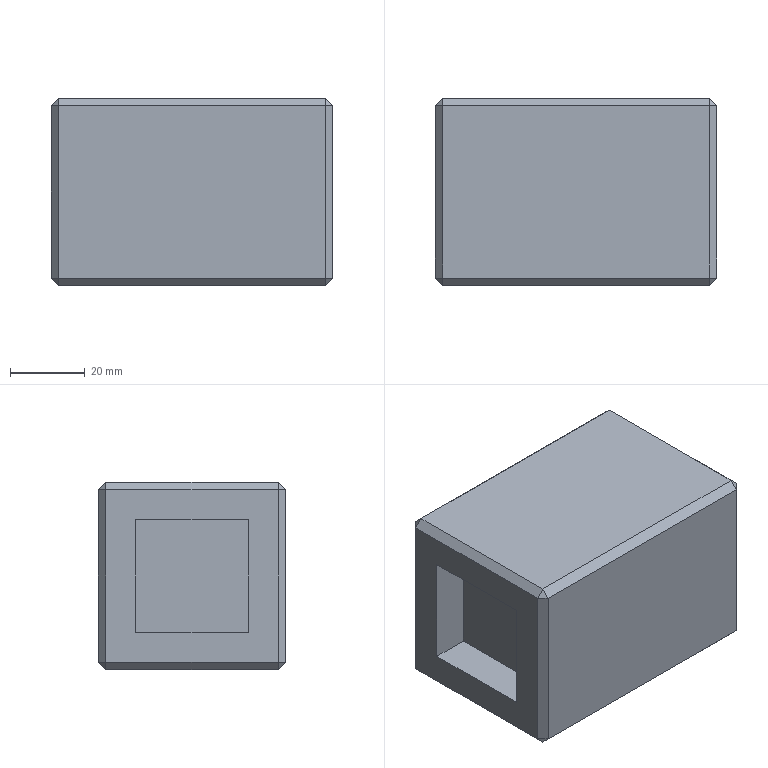Component | SolidWorks | ElectricalBox-2 | 1 solid | 36 faces | box 75 x 50 x 50 mm | volume 168143 mm3 | plane 36
build123d program:
from build123d import *

# Parameters (mm, degrees)
SKETCH1_W           = 75
SKETCH1_H           = 50
BOSS_EXTRUDE1_DEPTH = 50
SHELL1_T            = -10
BOSS_EXTRUDE2_START = -10
SKETCH2_W           = 30
SKETCH2_H           = 30
BOSS_EXTRUDE2_DEPTH = 55
CHAMFER1_SIZE       = 2


with BuildPart() as part:
    # Sketch1 → Boss-Extrude1 (new body)
    with BuildSketch(Plane.XY):
        with Locations((-82.5, 65)):
            Rectangle(SKETCH1_W, SKETCH1_H)
    extrude(amount=BOSS_EXTRUDE1_DEPTH)

    # Shell1
    shell1_openings = [part.faces().sort_by_distance(p)[0] for p in [
        (-120, 65, 25),
        (-45, 65, 25),
    ]]
    offset(amount=SHELL1_T, openings=shell1_openings, kind=Kind.INTERSECTION)

    # Sketch2 → Boss-Extrude2 (add)
    with BuildSketch(Plane.ZY.offset(120).offset(BOSS_EXTRUDE2_START)):
        with Locations((25, 65)):
            Rectangle(SKETCH2_W, SKETCH2_H)
    extrude(amount=-BOSS_EXTRUDE2_DEPTH)

    # Chamfer1
    chamfer1_edges = [part.edges().sort_by_distance(p)[0] for p in [
        (-120, 65, 50),
        (-82.5, 40, 50),
        (-45, 65, 50),
        (-82.5, 40, 0),
        (-120, 65, 0),
        (-82.5, 90, 0),
        (-45, 65, 0),
        (-45, 40, 25),
        (-120, 40, 25),
        (-120, 90, 25),
        (-45, 90, 25),
        (-82.5, 90, 50),
    ]]
    chamfer(chamfer1_edges, length=CHAMFER1_SIZE)


solid = part.part

# Placed as in the assembly
solid = solid.moved(Location((-690, 115, -100), (0, 0, 0)))
STEP:
#1=CARTESIAN_POINT('',(-31.496,6.496,-3.543));
#2=VERTEX_POINT('',#1);
#3=CARTESIAN_POINT('',(-31.89,6.496,-3.543));
#4=VERTEX_POINT('',#3);
#5=CARTESIAN_POINT('',(-27.165,6.496,-3.543));
#6=DIRECTION('',(-1.,0.,0.));
#7=VECTOR('',#6,39.37);
#8=LINE('',#5,#7);
#9=EDGE_CURVE('',#2,#4,#8,.T.);
#10=ORIENTED_EDGE('',*,*,#9,.F.);
#11=CARTESIAN_POINT('',(-31.496,7.677,-3.543));
#12=VERTEX_POINT('',#11);
#13=CARTESIAN_POINT('',(-31.496,7.677,-3.543));
#14=DIRECTION('',(0.,-1.,0.));
#15=VECTOR('',#14,39.37);
#16=LINE('',#13,#15);
#17=EDGE_CURVE('',#12,#2,#16,.T.);
#18=ORIENTED_EDGE('',*,*,#17,.F.);
#19=CARTESIAN_POINT('',(-31.89,7.677,-3.543));
#20=VERTEX_POINT('',#19);
#21=CARTESIAN_POINT('',(-27.165,7.677,-3.543));
#22=DIRECTION('',(-1.,0.,0.));
#23=VECTOR('',#22,39.37);
#24=LINE('',#21,#23);
#25=EDGE_CURVE('',#12,#20,#24,.T.);
#26=ORIENTED_EDGE('',*,*,#25,.T.);
#27=CARTESIAN_POINT('',(-31.89,8.071,-3.543));
#28=DIRECTION('',(0.,-1.,0.));
#29=VECTOR('',#28,39.37);
#30=LINE('',#27,#29);
#31=EDGE_CURVE('',#20,#4,#30,.T.);
#32=ORIENTED_EDGE('',*,*,#31,.T.);
#33=EDGE_LOOP('',(#10,#18,#26,#32));
#34=FACE_OUTER_BOUND('',#33,.T.);
#35=CARTESIAN_POINT('',(-28.937,8.071,-3.543));
#36=DIRECTION('',(0.,0.,1.));
#37=DIRECTION('',(0.,-1.,0.));
#38=AXIS2_PLACEMENT_3D('',#35,#36,#37);
#39=PLANE('',#38);
#40=ADVANCED_FACE('',(#34),#39,.T.);
#41=CARTESIAN_POINT('',(-31.89,7.677,-2.362));
#42=VERTEX_POINT('',#41);
#43=CARTESIAN_POINT('',(-31.496,7.677,-2.362));
#44=VERTEX_POINT('',#43);
#45=CARTESIAN_POINT('',(-27.165,7.677,-2.362));
#46=DIRECTION('',(1.,0.,0.));
#47=VECTOR('',#46,39.37);
#48=LINE('',#45,#47);
#49=EDGE_CURVE('',#42,#44,#48,.T.);
#50=ORIENTED_EDGE('',*,*,#49,.T.);
#51=CARTESIAN_POINT('',(-31.496,6.496,-2.362));
#52=VERTEX_POINT('',#51);
#53=CARTESIAN_POINT('',(-31.496,7.677,-2.362));
#54=DIRECTION('',(0.,1.,0.));
#55=VECTOR('',#54,39.37);
#56=LINE('',#53,#55);
#57=EDGE_CURVE('',#52,#44,#56,.T.);
#58=ORIENTED_EDGE('',*,*,#57,.F.);
#59=CARTESIAN_POINT('',(-31.89,6.496,-2.362));
#60=VERTEX_POINT('',#59);
#61=CARTESIAN_POINT('',(-27.165,6.496,-2.362));
#62=DIRECTION('',(1.,0.,0.));
#63=VECTOR('',#62,39.37);
#64=LINE('',#61,#63);
#65=EDGE_CURVE('',#60,#52,#64,.T.);
#66=ORIENTED_EDGE('',*,*,#65,.F.);
#67=CARTESIAN_POINT('',(-31.89,8.071,-2.362));
#68=DIRECTION('',(0.,-1.,0.));
#69=VECTOR('',#68,39.37);
#70=LINE('',#67,#69);
#71=EDGE_CURVE('',#42,#60,#70,.T.);
#72=ORIENTED_EDGE('',*,*,#71,.F.);
#73=EDGE_LOOP('',(#50,#58,#66,#72));
#74=FACE_OUTER_BOUND('',#73,.T.);
#75=CARTESIAN_POINT('',(-28.937,8.071,-2.362));
#76=DIRECTION('',(0.,0.,-1.));
#77=DIRECTION('',(0.,1.,0.));
#78=AXIS2_PLACEMENT_3D('',#75,#76,#77);
#79=PLANE('',#78);
#80=ADVANCED_FACE('',(#74),#79,.T.);
#81=ORIENTED_EDGE('',*,*,#25,.F.);
#82=CARTESIAN_POINT('',(-31.496,7.677,-3.543));
#83=DIRECTION('',(0.,0.,-1.));
#84=VECTOR('',#83,39.37);
#85=LINE('',#82,#84);
#86=EDGE_CURVE('',#44,#12,#85,.T.);
#87=ORIENTED_EDGE('',*,*,#86,.F.);
#88=ORIENTED_EDGE('',*,*,#49,.F.);
#89=CARTESIAN_POINT('',(-31.89,7.677,-0.3937));
#90=DIRECTION('',(0.,0.,1.));
#91=VECTOR('',#90,39.37);
#92=LINE('',#89,#91);
#93=EDGE_CURVE('',#20,#42,#92,.T.);
#94=ORIENTED_EDGE('',*,*,#93,.F.);
#95=EDGE_LOOP('',(#81,#87,#88,#94));
#96=FACE_OUTER_BOUND('',#95,.T.);
#97=CARTESIAN_POINT('',(-27.165,7.677,-0.3937));
#98=DIRECTION('',(0.,-1.,0.));
#99=DIRECTION('',(-1.,0.,0.));
#100=AXIS2_PLACEMENT_3D('',#97,#98,#99);
#101=PLANE('',#100);
#102=ADVANCED_FACE('',(#96),#101,.T.);
#103=CARTESIAN_POINT('',(-31.496,6.496,-3.543));
#104=DIRECTION('',(0.,0.,1.));
#105=VECTOR('',#104,39.37);
#106=LINE('',#103,#105);
#107=EDGE_CURVE('',#2,#52,#106,.T.);
#108=ORIENTED_EDGE('',*,*,#107,.F.);
#109=ORIENTED_EDGE('',*,*,#9,.T.);
#110=CARTESIAN_POINT('',(-31.89,6.496,-0.3937));
#111=DIRECTION('',(0.,0.,1.));
#112=VECTOR('',#111,39.37);
#113=LINE('',#110,#112);
#114=EDGE_CURVE('',#4,#60,#113,.T.);
#115=ORIENTED_EDGE('',*,*,#114,.T.);
#116=ORIENTED_EDGE('',*,*,#65,.T.);
#117=EDGE_LOOP('',(#108,#109,#115,#116));
#118=FACE_OUTER_BOUND('',#117,.T.);
#119=CARTESIAN_POINT('',(-27.165,6.496,-0.3937));
#120=DIRECTION('',(0.,-1.,0.));
#121=DIRECTION('',(-1.,0.,0.));
#122=AXIS2_PLACEMENT_3D('',#119,#120,#121);
#123=PLANE('',#122);
#124=ADVANCED_FACE('',(#118),#123,.F.);
#125=CARTESIAN_POINT('',(-28.937,7.992,-2.047));
#126=VERTEX_POINT('',#125);
#127=CARTESIAN_POINT('',(-28.937,6.181,-2.047));
#128=VERTEX_POINT('',#127);
#129=CARTESIAN_POINT('',(-28.937,8.071,-2.047));
#130=DIRECTION('',(0.,-1.,0.));
#131=VECTOR('',#130,39.37);
#132=LINE('',#129,#131);
#133=EDGE_CURVE('',#126,#128,#132,.T.);
#134=ORIENTED_EDGE('',*,*,#133,.T.);
#135=CARTESIAN_POINT('',(-28.937,6.181,-3.858));
#136=VERTEX_POINT('',#135);
#137=CARTESIAN_POINT('',(-28.937,6.181,-3.937));
#138=DIRECTION('',(-0.,0.,-1.));
#139=VECTOR('',#138,39.37);
#140=LINE('',#137,#139);
#141=EDGE_CURVE('',#128,#136,#140,.T.);
#142=ORIENTED_EDGE('',*,*,#141,.T.);
#143=CARTESIAN_POINT('',(-28.937,7.992,-3.858));
#144=VERTEX_POINT('',#143);
#145=CARTESIAN_POINT('',(-28.937,8.071,-3.858));
#146=DIRECTION('',(0.,1.,0.));
#147=VECTOR('',#146,39.37);
#148=LINE('',#145,#147);
#149=EDGE_CURVE('',#136,#144,#148,.T.);
#150=ORIENTED_EDGE('',*,*,#149,.T.);
#151=CARTESIAN_POINT('',(-28.937,7.992,-3.937));
#152=DIRECTION('',(0.,0.,1.));
#153=VECTOR('',#152,39.37);
#154=LINE('',#151,#153);
#155=EDGE_CURVE('',#144,#126,#154,.T.);
#156=ORIENTED_EDGE('',*,*,#155,.T.);
#157=EDGE_LOOP('',(#134,#142,#150,#156));
#158=FACE_OUTER_BOUND('',#157,.T.);
#159=CARTESIAN_POINT('',(-28.937,6.496,-2.362));
#160=VERTEX_POINT('',#159);
#161=CARTESIAN_POINT('',(-28.937,6.496,-3.543));
#162=VERTEX_POINT('',#161);
#163=CARTESIAN_POINT('',(-28.937,6.496,-0.3937));
#164=DIRECTION('',(-0.,0.,-1.));
#165=VECTOR('',#164,39.37);
#166=LINE('',#163,#165);
#167=EDGE_CURVE('',#160,#162,#166,.T.);
#168=ORIENTED_EDGE('',*,*,#167,.F.);
#169=CARTESIAN_POINT('',(-28.937,7.677,-2.362));
#170=VERTEX_POINT('',#169);
#171=CARTESIAN_POINT('',(-28.937,8.071,-2.362));
#172=DIRECTION('',(0.,-1.,0.));
#173=VECTOR('',#172,39.37);
#174=LINE('',#171,#173);
#175=EDGE_CURVE('',#170,#160,#174,.T.);
#176=ORIENTED_EDGE('',*,*,#175,.F.);
#177=CARTESIAN_POINT('',(-28.937,7.677,-3.543));
#178=VERTEX_POINT('',#177);
#179=CARTESIAN_POINT('',(-28.937,7.677,-0.3937));
#180=DIRECTION('',(-0.,0.,-1.));
#181=VECTOR('',#180,39.37);
#182=LINE('',#179,#181);
#183=EDGE_CURVE('',#170,#178,#182,.T.);
#184=ORIENTED_EDGE('',*,*,#183,.T.);
#185=CARTESIAN_POINT('',(-28.937,8.071,-3.543));
#186=DIRECTION('',(0.,-1.,0.));
#187=VECTOR('',#186,39.37);
#188=LINE('',#185,#187);
#189=EDGE_CURVE('',#178,#162,#188,.T.);
#190=ORIENTED_EDGE('',*,*,#189,.T.);
#191=EDGE_LOOP('',(#168,#176,#184,#190));
#192=FACE_BOUND('',#191,.T.);
#193=CARTESIAN_POINT('',(-28.937,8.071,-3.937));
#194=DIRECTION('',(-1.,0.,0.));
#195=DIRECTION('',(0.,0.,1.));
#196=AXIS2_PLACEMENT_3D('',#193,#194,#195);
#197=PLANE('',#196);
#198=ADVANCED_FACE('',(#158,#192),#197,.F.);
#199=CARTESIAN_POINT('',(-31.89,7.992,-3.858));
#200=VERTEX_POINT('',#199);
#201=CARTESIAN_POINT('',(-31.89,6.181,-3.858));
#202=VERTEX_POINT('',#201);
#203=CARTESIAN_POINT('',(-31.89,8.071,-3.858));
#204=DIRECTION('',(0.,-1.,0.));
#205=VECTOR('',#204,39.37);
#206=LINE('',#203,#205);
#207=EDGE_CURVE('',#200,#202,#206,.T.);
#208=ORIENTED_EDGE('',*,*,#207,.T.);
#209=CARTESIAN_POINT('',(-31.89,6.181,-2.047));
#210=VERTEX_POINT('',#209);
#211=CARTESIAN_POINT('',(-31.89,6.181,-1.969));
#212=DIRECTION('',(0.,0.,1.));
#213=VECTOR('',#212,39.37);
#214=LINE('',#211,#213);
#215=EDGE_CURVE('',#202,#210,#214,.T.);
#216=ORIENTED_EDGE('',*,*,#215,.T.);
#217=CARTESIAN_POINT('',(-31.89,7.992,-2.047));
#218=VERTEX_POINT('',#217);
#219=CARTESIAN_POINT('',(-31.89,8.071,-2.047));
#220=DIRECTION('',(0.,1.,0.));
#221=VECTOR('',#220,39.37);
#222=LINE('',#219,#221);
#223=EDGE_CURVE('',#210,#218,#222,.T.);
#224=ORIENTED_EDGE('',*,*,#223,.T.);
#225=CARTESIAN_POINT('',(-31.89,7.992,-3.937));
#226=DIRECTION('',(0.,0.,-1.));
#227=VECTOR('',#226,39.37);
#228=LINE('',#225,#227);
#229=EDGE_CURVE('',#218,#200,#228,.T.);
#230=ORIENTED_EDGE('',*,*,#229,.T.);
#231=EDGE_LOOP('',(#208,#216,#224,#230));
#232=FACE_OUTER_BOUND('',#231,.T.);
#233=ORIENTED_EDGE('',*,*,#114,.F.);
#234=ORIENTED_EDGE('',*,*,#31,.F.);
#235=ORIENTED_EDGE('',*,*,#93,.T.);
#236=ORIENTED_EDGE('',*,*,#71,.T.);
#237=EDGE_LOOP('',(#233,#234,#235,#236));
#238=FACE_BOUND('',#237,.T.);
#239=CARTESIAN_POINT('',(-31.89,8.071,-3.937));
#240=DIRECTION('',(1.,0.,0.));
#241=DIRECTION('',(0.,-1.,0.));
#242=AXIS2_PLACEMENT_3D('',#239,#240,#241);
#243=PLANE('',#242);
#244=ADVANCED_FACE('',(#232,#238),#243,.F.);
#245=CARTESIAN_POINT('',(-31.811,7.992,-3.937));
#246=VERTEX_POINT('',#245);
#247=CARTESIAN_POINT('',(-29.016,7.992,-3.937));
#248=VERTEX_POINT('',#247);
#249=CARTESIAN_POINT('',(-28.937,7.992,-3.937));
#250=DIRECTION('',(1.,0.,0.));
#251=VECTOR('',#250,39.37);
#252=LINE('',#249,#251);
#253=EDGE_CURVE('',#246,#248,#252,.T.);
#254=ORIENTED_EDGE('',*,*,#253,.T.);
#255=CARTESIAN_POINT('',(-29.016,6.181,-3.937));
#256=VERTEX_POINT('',#255);
#257=CARTESIAN_POINT('',(-29.016,8.071,-3.937));
#258=DIRECTION('',(0.,-1.,0.));
#259=VECTOR('',#258,39.37);
#260=LINE('',#257,#259);
#261=EDGE_CURVE('',#248,#256,#260,.T.);
#262=ORIENTED_EDGE('',*,*,#261,.T.);
#263=CARTESIAN_POINT('',(-31.811,6.181,-3.937));
#264=VERTEX_POINT('',#263);
#265=CARTESIAN_POINT('',(-31.89,6.181,-3.937));
#266=DIRECTION('',(-1.,0.,0.));
#267=VECTOR('',#266,39.37);
#268=LINE('',#265,#267);
#269=EDGE_CURVE('',#256,#264,#268,.T.);
#270=ORIENTED_EDGE('',*,*,#269,.T.);
#271=CARTESIAN_POINT('',(-31.811,8.071,-3.937));
#272=DIRECTION('',(0.,1.,0.));
#273=VECTOR('',#272,39.37);
#274=LINE('',#271,#273);
#275=EDGE_CURVE('',#264,#246,#274,.T.);
#276=ORIENTED_EDGE('',*,*,#275,.T.);
#277=EDGE_LOOP('',(#254,#262,#270,#276));
#278=FACE_OUTER_BOUND('',#277,.T.);
#279=CARTESIAN_POINT('',(-28.937,8.071,-3.937));
#280=DIRECTION('',(0.,0.,1.));
#281=DIRECTION('',(0.,-1.,0.));
#282=AXIS2_PLACEMENT_3D('',#279,#280,#281);
#283=PLANE('',#282);
#284=ADVANCED_FACE('',(#278),#283,.F.);
#285=CARTESIAN_POINT('',(-29.016,7.992,-1.969));
#286=VERTEX_POINT('',#285);
#287=CARTESIAN_POINT('',(-31.811,7.992,-1.969));
#288=VERTEX_POINT('',#287);
#289=CARTESIAN_POINT('',(-28.937,7.992,-1.969));
#290=DIRECTION('',(-1.,0.,0.));
#291=VECTOR('',#290,39.37);
#292=LINE('',#289,#291);
#293=EDGE_CURVE('',#286,#288,#292,.T.);
#294=ORIENTED_EDGE('',*,*,#293,.T.);
#295=CARTESIAN_POINT('',(-31.811,6.181,-1.969));
#296=VERTEX_POINT('',#295);
#297=CARTESIAN_POINT('',(-31.811,8.071,-1.969));
#298=DIRECTION('',(0.,-1.,0.));
#299=VECTOR('',#298,39.37);
#300=LINE('',#297,#299);
#301=EDGE_CURVE('',#288,#296,#300,.T.);
#302=ORIENTED_EDGE('',*,*,#301,.T.);
#303=CARTESIAN_POINT('',(-29.016,6.181,-1.969));
#304=VERTEX_POINT('',#303);
#305=CARTESIAN_POINT('',(-28.937,6.181,-1.969));
#306=DIRECTION('',(1.,0.,0.));
#307=VECTOR('',#306,39.37);
#308=LINE('',#305,#307);
#309=EDGE_CURVE('',#296,#304,#308,.T.);
#310=ORIENTED_EDGE('',*,*,#309,.T.);
#311=CARTESIAN_POINT('',(-29.016,8.071,-1.969));
#312=DIRECTION('',(0.,1.,0.));
#313=VECTOR('',#312,39.37);
#314=LINE('',#311,#313);
#315=EDGE_CURVE('',#304,#286,#314,.T.);
#316=ORIENTED_EDGE('',*,*,#315,.T.);
#317=EDGE_LOOP('',(#294,#302,#310,#316));
#318=FACE_OUTER_BOUND('',#317,.T.);
#319=CARTESIAN_POINT('',(-28.937,8.071,-1.969));
#320=DIRECTION('',(0.,0.,-1.));
#321=DIRECTION('',(0.,1.,0.));
#322=AXIS2_PLACEMENT_3D('',#319,#320,#321);
#323=PLANE('',#322);
#324=ADVANCED_FACE('',(#318),#323,.F.);
#325=CARTESIAN_POINT('',(-29.016,8.071,-3.858));
#326=VERTEX_POINT('',#325);
#327=CARTESIAN_POINT('',(-31.811,8.071,-3.858));
#328=VERTEX_POINT('',#327);
#329=CARTESIAN_POINT('',(-27.165,8.071,-3.858));
#330=DIRECTION('',(-1.,0.,0.));
#331=VECTOR('',#330,39.37);
#332=LINE('',#329,#331);
#333=EDGE_CURVE('',#326,#328,#332,.T.);
#334=ORIENTED_EDGE('',*,*,#333,.T.);
#335=CARTESIAN_POINT('',(-31.811,8.071,-2.047));
#336=VERTEX_POINT('',#335);
#337=CARTESIAN_POINT('',(-31.811,8.071,-0.3937));
#338=DIRECTION('',(0.,0.,1.));
#339=VECTOR('',#338,39.37);
#340=LINE('',#337,#339);
#341=EDGE_CURVE('',#328,#336,#340,.T.);
#342=ORIENTED_EDGE('',*,*,#341,.T.);
#343=CARTESIAN_POINT('',(-29.016,8.071,-2.047));
#344=VERTEX_POINT('',#343);
#345=CARTESIAN_POINT('',(-27.165,8.071,-2.047));
#346=DIRECTION('',(1.,0.,0.));
#347=VECTOR('',#346,39.37);
#348=LINE('',#345,#347);
#349=EDGE_CURVE('',#336,#344,#348,.T.);
#350=ORIENTED_EDGE('',*,*,#349,.T.);
#351=CARTESIAN_POINT('',(-29.016,8.071,-0.3937));
#352=DIRECTION('',(-0.,0.,-1.));
#353=VECTOR('',#352,39.37);
#354=LINE('',#351,#353);
#355=EDGE_CURVE('',#344,#326,#354,.T.);
#356=ORIENTED_EDGE('',*,*,#355,.T.);
#357=EDGE_LOOP('',(#334,#342,#350,#356));
#358=FACE_OUTER_BOUND('',#357,.T.);
#359=CARTESIAN_POINT('',(-27.165,8.071,-0.3937));
#360=DIRECTION('',(0.,-1.,0.));
#361=DIRECTION('',(-1.,0.,0.));
#362=AXIS2_PLACEMENT_3D('',#359,#360,#361);
#363=PLANE('',#362);
#364=ADVANCED_FACE('',(#358),#363,.F.);
#365=CARTESIAN_POINT('',(-31.811,6.102,-2.047));
#366=VERTEX_POINT('',#365);
#367=CARTESIAN_POINT('',(-31.811,6.102,-3.858));
#368=VERTEX_POINT('',#367);
#369=CARTESIAN_POINT('',(-31.811,6.102,-3.937));
#370=DIRECTION('',(0.,0.,-1.));
#371=VECTOR('',#370,39.37);
#372=LINE('',#369,#371);
#373=EDGE_CURVE('',#366,#368,#372,.T.);
#374=ORIENTED_EDGE('',*,*,#373,.T.);
#375=CARTESIAN_POINT('',(-29.016,6.102,-3.858));
#376=VERTEX_POINT('',#375);
#377=CARTESIAN_POINT('',(-28.937,6.102,-3.858));
#378=DIRECTION('',(1.,0.,0.));
#379=VECTOR('',#378,39.37);
#380=LINE('',#377,#379);
#381=EDGE_CURVE('',#368,#376,#380,.T.);
#382=ORIENTED_EDGE('',*,*,#381,.T.);
#383=CARTESIAN_POINT('',(-29.016,6.102,-2.047));
#384=VERTEX_POINT('',#383);
#385=CARTESIAN_POINT('',(-29.016,6.102,-1.969));
#386=DIRECTION('',(0.,0.,1.));
#387=VECTOR('',#386,39.37);
#388=LINE('',#385,#387);
#389=EDGE_CURVE('',#376,#384,#388,.T.);
#390=ORIENTED_EDGE('',*,*,#389,.T.);
#391=CARTESIAN_POINT('',(-31.89,6.102,-2.047));
#392=DIRECTION('',(-1.,0.,0.));
#393=VECTOR('',#392,39.37);
#394=LINE('',#391,#393);
#395=EDGE_CURVE('',#384,#366,#394,.T.);
#396=ORIENTED_EDGE('',*,*,#395,.T.);
#397=EDGE_LOOP('',(#374,#382,#390,#396));
#398=FACE_OUTER_BOUND('',#397,.T.);
#399=CARTESIAN_POINT('',(-27.165,6.102,-0.3937));
#400=DIRECTION('',(0.,-1.,0.));
#401=DIRECTION('',(-1.,0.,0.));
#402=AXIS2_PLACEMENT_3D('',#399,#400,#401);
#403=PLANE('',#402);
#404=ADVANCED_FACE('',(#398),#403,.T.);
#405=CARTESIAN_POINT('',(-29.331,7.677,-3.543));
#406=VERTEX_POINT('',#405);
#407=CARTESIAN_POINT('',(-29.331,6.496,-3.543));
#408=VERTEX_POINT('',#407);
#409=CARTESIAN_POINT('',(-29.331,7.677,-3.543));
#410=DIRECTION('',(0.,-1.,0.));
#411=VECTOR('',#410,39.37);
#412=LINE('',#409,#411);
#413=EDGE_CURVE('',#406,#408,#412,.T.);
#414=ORIENTED_EDGE('',*,*,#413,.T.);
#415=CARTESIAN_POINT('',(-27.165,6.496,-3.543));
#416=DIRECTION('',(-1.,0.,0.));
#417=VECTOR('',#416,39.37);
#418=LINE('',#415,#417);
#419=EDGE_CURVE('',#162,#408,#418,.T.);
#420=ORIENTED_EDGE('',*,*,#419,.F.);
#421=ORIENTED_EDGE('',*,*,#189,.F.);
#422=CARTESIAN_POINT('',(-27.165,7.677,-3.543));
#423=DIRECTION('',(-1.,0.,0.));
#424=VECTOR('',#423,39.37);
#425=LINE('',#422,#424);
#426=EDGE_CURVE('',#178,#406,#425,.T.);
#427=ORIENTED_EDGE('',*,*,#426,.T.);
#428=EDGE_LOOP('',(#414,#420,#421,#427));
#429=FACE_OUTER_BOUND('',#428,.T.);
#430=CARTESIAN_POINT('',(-28.937,8.071,-3.543));
#431=DIRECTION('',(0.,0.,1.));
#432=DIRECTION('',(0.,-1.,0.));
#433=AXIS2_PLACEMENT_3D('',#430,#431,#432);
#434=PLANE('',#433);
#435=ADVANCED_FACE('',(#429),#434,.T.);
#436=CARTESIAN_POINT('',(-29.331,6.496,-2.362));
#437=VERTEX_POINT('',#436);
#438=CARTESIAN_POINT('',(-29.331,7.677,-2.362));
#439=VERTEX_POINT('',#438);
#440=CARTESIAN_POINT('',(-29.331,7.677,-2.362));
#441=DIRECTION('',(0.,1.,0.));
#442=VECTOR('',#441,39.37);
#443=LINE('',#440,#442);
#444=EDGE_CURVE('',#437,#439,#443,.T.);
#445=ORIENTED_EDGE('',*,*,#444,.T.);
#446=CARTESIAN_POINT('',(-27.165,7.677,-2.362));
#447=DIRECTION('',(1.,0.,0.));
#448=VECTOR('',#447,39.37);
#449=LINE('',#446,#448);
#450=EDGE_CURVE('',#439,#170,#449,.T.);
#451=ORIENTED_EDGE('',*,*,#450,.T.);
#452=ORIENTED_EDGE('',*,*,#175,.T.);
#453=CARTESIAN_POINT('',(-27.165,6.496,-2.362));
#454=DIRECTION('',(1.,0.,0.));
#455=VECTOR('',#454,39.37);
#456=LINE('',#453,#455);
#457=EDGE_CURVE('',#437,#160,#456,.T.);
#458=ORIENTED_EDGE('',*,*,#457,.F.);
#459=EDGE_LOOP('',(#445,#451,#452,#458));
#460=FACE_OUTER_BOUND('',#459,.T.);
#461=CARTESIAN_POINT('',(-28.937,8.071,-2.362));
#462=DIRECTION('',(0.,0.,-1.));
#463=DIRECTION('',(0.,1.,0.));
#464=AXIS2_PLACEMENT_3D('',#461,#462,#463);
#465=PLANE('',#464);
#466=ADVANCED_FACE('',(#460),#465,.T.);
#467=CARTESIAN_POINT('',(-29.331,7.677,-3.543));
#468=DIRECTION('',(0.,0.,-1.));
#469=VECTOR('',#468,39.37);
#470=LINE('',#467,#469);
#471=EDGE_CURVE('',#439,#406,#470,.T.);
#472=ORIENTED_EDGE('',*,*,#471,.T.);
#473=ORIENTED_EDGE('',*,*,#426,.F.);
#474=ORIENTED_EDGE('',*,*,#183,.F.);
#475=ORIENTED_EDGE('',*,*,#450,.F.);
#476=EDGE_LOOP('',(#472,#473,#474,#475));
#477=FACE_OUTER_BOUND('',#476,.T.);
#478=CARTESIAN_POINT('',(-27.165,7.677,-0.3937));
#479=DIRECTION('',(0.,-1.,0.));
#480=DIRECTION('',(-1.,0.,0.));
#481=AXIS2_PLACEMENT_3D('',#478,#479,#480);
#482=PLANE('',#481);
#483=ADVANCED_FACE('',(#477),#482,.T.);
#484=ORIENTED_EDGE('',*,*,#419,.T.);
#485=CARTESIAN_POINT('',(-29.331,6.496,-3.543));
#486=DIRECTION('',(0.,0.,1.));
#487=VECTOR('',#486,39.37);
#488=LINE('',#485,#487);
#489=EDGE_CURVE('',#408,#437,#488,.T.);
#490=ORIENTED_EDGE('',*,*,#489,.T.);
#491=ORIENTED_EDGE('',*,*,#457,.T.);
#492=ORIENTED_EDGE('',*,*,#167,.T.);
#493=EDGE_LOOP('',(#484,#490,#491,#492));
#494=FACE_OUTER_BOUND('',#493,.T.);
#495=CARTESIAN_POINT('',(-27.165,6.496,-0.3937));
#496=DIRECTION('',(0.,-1.,0.));
#497=DIRECTION('',(-1.,0.,0.));
#498=AXIS2_PLACEMENT_3D('',#495,#496,#497);
#499=PLANE('',#498);
#500=ADVANCED_FACE('',(#494),#499,.F.);
#501=ORIENTED_EDGE('',*,*,#86,.T.);
#502=ORIENTED_EDGE('',*,*,#17,.T.);
#503=ORIENTED_EDGE('',*,*,#107,.T.);
#504=ORIENTED_EDGE('',*,*,#57,.T.);
#505=EDGE_LOOP('',(#501,#502,#503,#504));
#506=FACE_OUTER_BOUND('',#505,.T.);
#507=CARTESIAN_POINT('',(-31.496,6.102,-0.3937));
#508=DIRECTION('',(1.,0.,0.));
#509=DIRECTION('',(0.,-1.,0.));
#510=AXIS2_PLACEMENT_3D('',#507,#508,#509);
#511=PLANE('',#510);
#512=ADVANCED_FACE('',(#506),#511,.F.);
#513=ORIENTED_EDGE('',*,*,#471,.F.);
#514=ORIENTED_EDGE('',*,*,#444,.F.);
#515=ORIENTED_EDGE('',*,*,#489,.F.);
#516=ORIENTED_EDGE('',*,*,#413,.F.);
#517=EDGE_LOOP('',(#513,#514,#515,#516));
#518=FACE_OUTER_BOUND('',#517,.T.);
#519=CARTESIAN_POINT('',(-29.331,6.102,-0.3937));
#520=DIRECTION('',(1.,0.,0.));
#521=DIRECTION('',(0.,-1.,0.));
#522=AXIS2_PLACEMENT_3D('',#519,#520,#521);
#523=PLANE('',#522);
#524=ADVANCED_FACE('',(#518),#523,.T.);
#525=CARTESIAN_POINT('',(-28.937,7.992,-3.858));
#526=DIRECTION('',(0.7071,-0.7071,0.));
#527=VECTOR('',#526,39.37);
#528=LINE('',#525,#527);
#529=EDGE_CURVE('',#326,#144,#528,.T.);
#530=ORIENTED_EDGE('',*,*,#529,.F.);
#531=ORIENTED_EDGE('',*,*,#355,.F.);
#532=CARTESIAN_POINT('',(-28.937,7.992,-2.047));
#533=DIRECTION('',(-0.7071,0.7071,-0.));
#534=VECTOR('',#533,39.37);
#535=LINE('',#532,#534);
#536=EDGE_CURVE('',#126,#344,#535,.T.);
#537=ORIENTED_EDGE('',*,*,#536,.F.);
#538=ORIENTED_EDGE('',*,*,#155,.F.);
#539=EDGE_LOOP('',(#530,#531,#537,#538));
#540=FACE_OUTER_BOUND('',#539,.T.);
#541=CARTESIAN_POINT('',(-29.016,8.071,-0.3937));
#542=DIRECTION('',(-0.7071,-0.7071,0.));
#543=DIRECTION('',(-0.,0.,-1.));
#544=AXIS2_PLACEMENT_3D('',#541,#542,#543);
#545=PLANE('',#544);
#546=ADVANCED_FACE('',(#540),#545,.F.);
#547=CARTESIAN_POINT('',(-29.016,8.031,-3.898));
#548=DIRECTION('',(-0.,-0.7071,-0.7071));
#549=VECTOR('',#548,39.37);
#550=LINE('',#547,#549);
#551=EDGE_CURVE('',#326,#248,#550,.T.);
#552=ORIENTED_EDGE('',*,*,#551,.F.);
#553=ORIENTED_EDGE('',*,*,#529,.T.);
#554=CARTESIAN_POINT('',(-28.937,7.992,-3.858));
#555=DIRECTION('',(0.7071,-0.,0.7071));
#556=VECTOR('',#555,39.37);
#557=LINE('',#554,#556);
#558=EDGE_CURVE('',#248,#144,#557,.T.);
#559=ORIENTED_EDGE('',*,*,#558,.F.);
#560=EDGE_LOOP('',(#552,#553,#559));
#561=FACE_OUTER_BOUND('',#560,.T.);
#562=CARTESIAN_POINT('',(-28.937,7.992,-3.858));
#563=DIRECTION('',(0.5774,0.5774,-0.5774));
#564=DIRECTION('',(-0.7071,0.,-0.7071));
#565=AXIS2_PLACEMENT_3D('',#562,#563,#564);
#566=PLANE('',#565);
#567=ADVANCED_FACE('',(#561),#566,.T.);
#568=CARTESIAN_POINT('',(-28.937,7.992,-2.047));
#569=DIRECTION('',(-0.7071,0.,0.7071));
#570=VECTOR('',#569,39.37);
#571=LINE('',#568,#570);
#572=EDGE_CURVE('',#126,#286,#571,.T.);
#573=ORIENTED_EDGE('',*,*,#572,.F.);
#574=ORIENTED_EDGE('',*,*,#536,.T.);
#575=CARTESIAN_POINT('',(-29.016,8.031,-2.008));
#576=DIRECTION('',(-0.,0.7071,-0.7071));
#577=VECTOR('',#576,39.37);
#578=LINE('',#575,#577);
#579=EDGE_CURVE('',#286,#344,#578,.T.);
#580=ORIENTED_EDGE('',*,*,#579,.F.);
#581=EDGE_LOOP('',(#573,#574,#580));
#582=FACE_OUTER_BOUND('',#581,.T.);
#583=CARTESIAN_POINT('',(-28.937,7.992,-2.047));
#584=DIRECTION('',(0.5774,0.5774,0.5774));
#585=DIRECTION('',(0.7071,-0.7071,0.));
#586=AXIS2_PLACEMENT_3D('',#583,#584,#585);
#587=PLANE('',#586);
#588=ADVANCED_FACE('',(#582),#587,.T.);
#589=ORIENTED_EDGE('',*,*,#558,.T.);
#590=ORIENTED_EDGE('',*,*,#149,.F.);
#591=CARTESIAN_POINT('',(-28.937,6.181,-3.858));
#592=DIRECTION('',(0.7071,0.,0.7071));
#593=VECTOR('',#592,39.37);
#594=LINE('',#591,#593);
#595=EDGE_CURVE('',#256,#136,#594,.T.);
#596=ORIENTED_EDGE('',*,*,#595,.F.);
#597=ORIENTED_EDGE('',*,*,#261,.F.);
#598=EDGE_LOOP('',(#589,#590,#596,#597));
#599=FACE_OUTER_BOUND('',#598,.T.);
#600=CARTESIAN_POINT('',(-29.016,8.071,-3.937));
#601=DIRECTION('',(-0.7071,0.,0.7071));
#602=DIRECTION('',(0.,-1.,0.));
#603=AXIS2_PLACEMENT_3D('',#600,#601,#602);
#604=PLANE('',#603);
#605=ADVANCED_FACE('',(#599),#604,.F.);
#606=ORIENTED_EDGE('',*,*,#551,.T.);
#607=ORIENTED_EDGE('',*,*,#253,.F.);
#608=CARTESIAN_POINT('',(-31.811,7.992,-3.937));
#609=DIRECTION('',(0.,-0.7071,-0.7071));
#610=VECTOR('',#609,39.37);
#611=LINE('',#608,#610);
#612=EDGE_CURVE('',#328,#246,#611,.T.);
#613=ORIENTED_EDGE('',*,*,#612,.F.);
#614=ORIENTED_EDGE('',*,*,#333,.F.);
#615=EDGE_LOOP('',(#606,#607,#613,#614));
#616=FACE_OUTER_BOUND('',#615,.T.);
#617=CARTESIAN_POINT('',(-27.165,8.071,-3.858));
#618=DIRECTION('',(0.,-0.7071,0.7071));
#619=DIRECTION('',(-1.,0.,0.));
#620=AXIS2_PLACEMENT_3D('',#617,#618,#619);
#621=PLANE('',#620);
#622=ADVANCED_FACE('',(#616),#621,.F.);
#623=CARTESIAN_POINT('',(-31.811,8.071,-2.047));
#624=DIRECTION('',(-0.7071,-0.7071,-0.));
#625=VECTOR('',#624,39.37);
#626=LINE('',#623,#625);
#627=EDGE_CURVE('',#336,#218,#626,.T.);
#628=ORIENTED_EDGE('',*,*,#627,.F.);
#629=ORIENTED_EDGE('',*,*,#341,.F.);
#630=CARTESIAN_POINT('',(-31.85,8.031,-3.858));
#631=DIRECTION('',(0.7071,0.7071,-0.));
#632=VECTOR('',#631,39.37);
#633=LINE('',#630,#632);
#634=EDGE_CURVE('',#200,#328,#633,.T.);
#635=ORIENTED_EDGE('',*,*,#634,.F.);
#636=ORIENTED_EDGE('',*,*,#229,.F.);
#637=EDGE_LOOP('',(#628,#629,#635,#636));
#638=FACE_OUTER_BOUND('',#637,.T.);
#639=CARTESIAN_POINT('',(-31.811,8.071,-0.3937));
#640=DIRECTION('',(0.7071,-0.7071,0.));
#641=DIRECTION('',(0.,0.,1.));
#642=AXIS2_PLACEMENT_3D('',#639,#640,#641);
#643=PLANE('',#642);
#644=ADVANCED_FACE('',(#638),#643,.F.);
#645=ORIENTED_EDGE('',*,*,#579,.T.);
#646=ORIENTED_EDGE('',*,*,#349,.F.);
#647=CARTESIAN_POINT('',(-31.811,8.071,-2.047));
#648=DIRECTION('',(0.,0.7071,-0.7071));
#649=VECTOR('',#648,39.37);
#650=LINE('',#647,#649);
#651=EDGE_CURVE('',#288,#336,#650,.T.);
#652=ORIENTED_EDGE('',*,*,#651,.F.);
#653=ORIENTED_EDGE('',*,*,#293,.F.);
#654=EDGE_LOOP('',(#645,#646,#652,#653));
#655=FACE_OUTER_BOUND('',#654,.T.);
#656=CARTESIAN_POINT('',(-27.165,8.071,-2.047));
#657=DIRECTION('',(0.,-0.7071,-0.7071));
#658=DIRECTION('',(1.,0.,0.));
#659=AXIS2_PLACEMENT_3D('',#656,#657,#658);
#660=PLANE('',#659);
#661=ADVANCED_FACE('',(#655),#660,.F.);
#662=ORIENTED_EDGE('',*,*,#572,.T.);
#663=ORIENTED_EDGE('',*,*,#315,.F.);
#664=CARTESIAN_POINT('',(-28.976,6.181,-2.008));
#665=DIRECTION('',(-0.7071,-0.,0.7071));
#666=VECTOR('',#665,39.37);
#667=LINE('',#664,#666);
#668=EDGE_CURVE('',#128,#304,#667,.T.);
#669=ORIENTED_EDGE('',*,*,#668,.F.);
#670=ORIENTED_EDGE('',*,*,#133,.F.);
#671=EDGE_LOOP('',(#662,#663,#669,#670));
#672=FACE_OUTER_BOUND('',#671,.T.);
#673=CARTESIAN_POINT('',(-28.937,8.071,-2.047));
#674=DIRECTION('',(-0.7071,0.,-0.7071));
#675=DIRECTION('',(0.,-1.,0.));
#676=AXIS2_PLACEMENT_3D('',#673,#674,#675);
#677=PLANE('',#676);
#678=ADVANCED_FACE('',(#672),#677,.F.);
#679=CARTESIAN_POINT('',(-28.937,6.181,-3.858));
#680=DIRECTION('',(-0.7071,-0.7071,0.));
#681=VECTOR('',#680,39.37);
#682=LINE('',#679,#681);
#683=EDGE_CURVE('',#136,#376,#682,.T.);
#684=ORIENTED_EDGE('',*,*,#683,.F.);
#685=ORIENTED_EDGE('',*,*,#141,.F.);
#686=CARTESIAN_POINT('',(-29.016,6.102,-2.047));
#687=DIRECTION('',(0.7071,0.7071,0.));
#688=VECTOR('',#687,39.37);
#689=LINE('',#686,#688);
#690=EDGE_CURVE('',#384,#128,#689,.T.);
#691=ORIENTED_EDGE('',*,*,#690,.F.);
#692=ORIENTED_EDGE('',*,*,#389,.F.);
#693=EDGE_LOOP('',(#684,#685,#691,#692));
#694=FACE_OUTER_BOUND('',#693,.T.);
#695=CARTESIAN_POINT('',(-28.937,6.181,-3.937));
#696=DIRECTION('',(0.7071,-0.7071,-0.));
#697=DIRECTION('',(0.,0.,1.));
#698=AXIS2_PLACEMENT_3D('',#695,#696,#697);
#699=PLANE('',#698);
#700=ADVANCED_FACE('',(#694),#699,.T.);
#701=ORIENTED_EDGE('',*,*,#595,.T.);
#702=ORIENTED_EDGE('',*,*,#683,.T.);
#703=CARTESIAN_POINT('',(-29.016,6.142,-3.898));
#704=DIRECTION('',(-0.,-0.7071,0.7071));
#705=VECTOR('',#704,39.37);
#706=LINE('',#703,#705);
#707=EDGE_CURVE('',#256,#376,#706,.T.);
#708=ORIENTED_EDGE('',*,*,#707,.F.);
#709=EDGE_LOOP('',(#701,#702,#708));
#710=FACE_OUTER_BOUND('',#709,.T.);
#711=CARTESIAN_POINT('',(-28.937,6.181,-3.858));
#712=DIRECTION('',(0.5774,-0.5774,-0.5774));
#713=DIRECTION('',(-0.7071,-0.7071,0.));
#714=AXIS2_PLACEMENT_3D('',#711,#712,#713);
#715=PLANE('',#714);
#716=ADVANCED_FACE('',(#710),#715,.T.);
#717=ORIENTED_EDGE('',*,*,#634,.T.);
#718=ORIENTED_EDGE('',*,*,#612,.T.);
#719=CARTESIAN_POINT('',(-31.811,7.992,-3.937));
#720=DIRECTION('',(0.7071,-0.,-0.7071));
#721=VECTOR('',#720,39.37);
#722=LINE('',#719,#721);
#723=EDGE_CURVE('',#200,#246,#722,.T.);
#724=ORIENTED_EDGE('',*,*,#723,.F.);
#725=EDGE_LOOP('',(#717,#718,#724));
#726=FACE_OUTER_BOUND('',#725,.T.);
#727=CARTESIAN_POINT('',(-31.811,7.992,-3.937));
#728=DIRECTION('',(-0.5774,0.5774,-0.5774));
#729=DIRECTION('',(-0.7071,0.,0.7071));
#730=AXIS2_PLACEMENT_3D('',#727,#728,#729);
#731=PLANE('',#730);
#732=ADVANCED_FACE('',(#726),#731,.T.);
#733=ORIENTED_EDGE('',*,*,#651,.T.);
#734=ORIENTED_EDGE('',*,*,#627,.T.);
#735=CARTESIAN_POINT('',(-31.85,7.992,-2.008));
#736=DIRECTION('',(-0.7071,-0.,-0.7071));
#737=VECTOR('',#736,39.37);
#738=LINE('',#735,#737);
#739=EDGE_CURVE('',#288,#218,#738,.T.);
#740=ORIENTED_EDGE('',*,*,#739,.F.);
#741=EDGE_LOOP('',(#733,#734,#740));
#742=FACE_OUTER_BOUND('',#741,.T.);
#743=CARTESIAN_POINT('',(-31.811,8.071,-2.047));
#744=DIRECTION('',(-0.5774,0.5774,0.5774));
#745=DIRECTION('',(0.7071,0.7071,0.));
#746=AXIS2_PLACEMENT_3D('',#743,#744,#745);
#747=PLANE('',#746);
#748=ADVANCED_FACE('',(#742),#747,.T.);
#749=ORIENTED_EDGE('',*,*,#690,.T.);
#750=ORIENTED_EDGE('',*,*,#668,.T.);
#751=CARTESIAN_POINT('',(-29.016,6.102,-2.047));
#752=DIRECTION('',(0.,0.7071,0.7071));
#753=VECTOR('',#752,39.37);
#754=LINE('',#751,#753);
#755=EDGE_CURVE('',#384,#304,#754,.T.);
#756=ORIENTED_EDGE('',*,*,#755,.F.);
#757=EDGE_LOOP('',(#749,#750,#756));
#758=FACE_OUTER_BOUND('',#757,.T.);
#759=CARTESIAN_POINT('',(-29.016,6.102,-2.047));
#760=DIRECTION('',(0.5774,-0.5774,0.5774));
#761=DIRECTION('',(-0.7071,-0.7071,0.));
#762=AXIS2_PLACEMENT_3D('',#759,#760,#761);
#763=PLANE('',#762);
#764=ADVANCED_FACE('',(#758),#763,.T.);
#765=ORIENTED_EDGE('',*,*,#707,.T.);
#766=ORIENTED_EDGE('',*,*,#381,.F.);
#767=CARTESIAN_POINT('',(-31.811,6.102,-3.858));
#768=DIRECTION('',(0.,-0.7071,0.7071));
#769=VECTOR('',#768,39.37);
#770=LINE('',#767,#769);
#771=EDGE_CURVE('',#264,#368,#770,.T.);
#772=ORIENTED_EDGE('',*,*,#771,.F.);
#773=ORIENTED_EDGE('',*,*,#269,.F.);
#774=EDGE_LOOP('',(#765,#766,#772,#773));
#775=FACE_OUTER_BOUND('',#774,.T.);
#776=CARTESIAN_POINT('',(-28.937,6.181,-3.937));
#777=DIRECTION('',(0.,-0.7071,-0.7071));
#778=DIRECTION('',(1.,0.,0.));
#779=AXIS2_PLACEMENT_3D('',#776,#777,#778);
#780=PLANE('',#779);
#781=ADVANCED_FACE('',(#775),#780,.T.);
#782=ORIENTED_EDGE('',*,*,#723,.T.);
#783=ORIENTED_EDGE('',*,*,#275,.F.);
#784=CARTESIAN_POINT('',(-31.85,6.181,-3.898));
#785=DIRECTION('',(0.7071,0.,-0.7071));
#786=VECTOR('',#785,39.37);
#787=LINE('',#784,#786);
#788=EDGE_CURVE('',#202,#264,#787,.T.);
#789=ORIENTED_EDGE('',*,*,#788,.F.);
#790=ORIENTED_EDGE('',*,*,#207,.F.);
#791=EDGE_LOOP('',(#782,#783,#789,#790));
#792=FACE_OUTER_BOUND('',#791,.T.);
#793=CARTESIAN_POINT('',(-31.89,8.071,-3.858));
#794=DIRECTION('',(0.7071,0.,0.7071));
#795=DIRECTION('',(0.,-1.,0.));
#796=AXIS2_PLACEMENT_3D('',#793,#794,#795);
#797=PLANE('',#796);
#798=ADVANCED_FACE('',(#792),#797,.F.);
#799=ORIENTED_EDGE('',*,*,#739,.T.);
#800=ORIENTED_EDGE('',*,*,#223,.F.);
#801=CARTESIAN_POINT('',(-31.89,6.181,-2.047));
#802=DIRECTION('',(-0.7071,0.,-0.7071));
#803=VECTOR('',#802,39.37);
#804=LINE('',#801,#803);
#805=EDGE_CURVE('',#296,#210,#804,.T.);
#806=ORIENTED_EDGE('',*,*,#805,.F.);
#807=ORIENTED_EDGE('',*,*,#301,.F.);
#808=EDGE_LOOP('',(#799,#800,#806,#807));
#809=FACE_OUTER_BOUND('',#808,.T.);
#810=CARTESIAN_POINT('',(-31.811,8.071,-1.969));
#811=DIRECTION('',(0.7071,0.,-0.7071));
#812=DIRECTION('',(0.,-1.,0.));
#813=AXIS2_PLACEMENT_3D('',#810,#811,#812);
#814=PLANE('',#813);
#815=ADVANCED_FACE('',(#809),#814,.F.);
#816=ORIENTED_EDGE('',*,*,#755,.T.);
#817=ORIENTED_EDGE('',*,*,#309,.F.);
#818=CARTESIAN_POINT('',(-31.811,6.142,-2.008));
#819=DIRECTION('',(-0.,0.7071,0.7071));
#820=VECTOR('',#819,39.37);
#821=LINE('',#818,#820);
#822=EDGE_CURVE('',#366,#296,#821,.T.);
#823=ORIENTED_EDGE('',*,*,#822,.F.);
#824=ORIENTED_EDGE('',*,*,#395,.F.);
#825=EDGE_LOOP('',(#816,#817,#823,#824));
#826=FACE_OUTER_BOUND('',#825,.T.);
#827=CARTESIAN_POINT('',(-28.937,6.181,-1.969));
#828=DIRECTION('',(0.,-0.7071,0.7071));
#829=DIRECTION('',(-1.,0.,0.));
#830=AXIS2_PLACEMENT_3D('',#827,#828,#829);
#831=PLANE('',#830);
#832=ADVANCED_FACE('',(#826),#831,.T.);
#833=ORIENTED_EDGE('',*,*,#788,.T.);
#834=ORIENTED_EDGE('',*,*,#771,.T.);
#835=CARTESIAN_POINT('',(-31.811,6.102,-3.858));
#836=DIRECTION('',(0.7071,-0.7071,0.));
#837=VECTOR('',#836,39.37);
#838=LINE('',#835,#837);
#839=EDGE_CURVE('',#202,#368,#838,.T.);
#840=ORIENTED_EDGE('',*,*,#839,.F.);
#841=EDGE_LOOP('',(#833,#834,#840));
#842=FACE_OUTER_BOUND('',#841,.T.);
#843=CARTESIAN_POINT('',(-31.811,6.102,-3.858));
#844=DIRECTION('',(-0.5774,-0.5774,-0.5774));
#845=DIRECTION('',(0.,0.7071,-0.7071));
#846=AXIS2_PLACEMENT_3D('',#843,#844,#845);
#847=PLANE('',#846);
#848=ADVANCED_FACE('',(#842),#847,.T.);
#849=ORIENTED_EDGE('',*,*,#822,.T.);
#850=ORIENTED_EDGE('',*,*,#805,.T.);
#851=CARTESIAN_POINT('',(-31.89,6.181,-2.047));
#852=DIRECTION('',(-0.7071,0.7071,0.));
#853=VECTOR('',#852,39.37);
#854=LINE('',#851,#853);
#855=EDGE_CURVE('',#366,#210,#854,.T.);
#856=ORIENTED_EDGE('',*,*,#855,.F.);
#857=EDGE_LOOP('',(#849,#850,#856));
#858=FACE_OUTER_BOUND('',#857,.T.);
#859=CARTESIAN_POINT('',(-31.89,6.181,-2.047));
#860=DIRECTION('',(-0.5774,-0.5774,0.5774));
#861=DIRECTION('',(-0.7071,0.7071,0.));
#862=AXIS2_PLACEMENT_3D('',#859,#860,#861);
#863=PLANE('',#862);
#864=ADVANCED_FACE('',(#858),#863,.T.);
#865=ORIENTED_EDGE('',*,*,#839,.T.);
#866=ORIENTED_EDGE('',*,*,#373,.F.);
#867=ORIENTED_EDGE('',*,*,#855,.T.);
#868=ORIENTED_EDGE('',*,*,#215,.F.);
#869=EDGE_LOOP('',(#865,#866,#867,#868));
#870=FACE_OUTER_BOUND('',#869,.T.);
#871=CARTESIAN_POINT('',(-31.89,6.181,-3.937));
#872=DIRECTION('',(-0.7071,-0.7071,0.));
#873=DIRECTION('',(0.,0.,-1.));
#874=AXIS2_PLACEMENT_3D('',#871,#872,#873);
#875=PLANE('',#874);
#876=ADVANCED_FACE('',(#870),#875,.T.);
#877=CLOSED_SHELL('',(#40,#80,#102,#124,#198,#244,#284,#324,#364,#404,#435,#466,#483,#500,#512,#524,#546,#567,#588,#605,#622,#644,#661,#678,#700,#716,#732,#748,#764,#781,#798,#815,#832,#848,#864,#876));
#878=MANIFOLD_SOLID_BREP('',#877);
#879=CARTESIAN_POINT('',(0.,0.,0.));
#880=DIRECTION('',(0.,0.,1.));
#881=DIRECTION('',(1.,0.,0.));
#882=AXIS2_PLACEMENT_3D('',#879,#880,#881);
#883=(LENGTH_UNIT()NAMED_UNIT(*)SI_UNIT($,.METRE.));
#884=LENGTH_MEASURE_WITH_UNIT(LENGTH_MEASURE(0.0254),#883);
#885=DIMENSIONAL_EXPONENTS(1.,0.,0.,0.,0.,0.,0.);
#886=(CONVERSION_BASED_UNIT('',#884)LENGTH_UNIT()NAMED_UNIT(#885));
#887=UNCERTAINTY_MEASURE_WITH_UNIT(LENGTH_MEASURE(0.00001),#886,'','');
#888=(NAMED_UNIT(*)PLANE_ANGLE_UNIT()SI_UNIT($,.RADIAN.));
#889=(NAMED_UNIT(*)SI_UNIT($,.STERADIAN.)SOLID_ANGLE_UNIT());
#890=(GEOMETRIC_REPRESENTATION_CONTEXT(3)GLOBAL_UNCERTAINTY_ASSIGNED_CONTEXT((#887))GLOBAL_UNIT_ASSIGNED_CONTEXT((#886,#888,#889))REPRESENTATION_CONTEXT('',''));
#891=ADVANCED_BREP_SHAPE_REPRESENTATION('',(#878,#882),#890);
#892=COLOUR_RGB('',0.7922,0.8196,0.9333);
#893=FILL_AREA_STYLE_COLOUR('',#892);
#894=FILL_AREA_STYLE('',(#893));
#895=SURFACE_STYLE_FILL_AREA(#894);
#896=SURFACE_SIDE_STYLE('',(#895));
#897=SURFACE_STYLE_USAGE(.BOTH.,#896);
#898=PRESENTATION_STYLE_ASSIGNMENT((#897));
#899=STYLED_ITEM('',(#898),#878);
#900=PRESENTATION_LAYER_ASSIGNMENT('','',(#899));
#901=(LENGTH_UNIT()NAMED_UNIT(*)SI_UNIT($,.METRE.));
#902=LENGTH_MEASURE_WITH_UNIT(LENGTH_MEASURE(0.0254),#901);
#903=DIMENSIONAL_EXPONENTS(1.,0.,0.,0.,0.,0.,0.);
#904=(CONVERSION_BASED_UNIT('',#902)LENGTH_UNIT()NAMED_UNIT(#903));
#905=UNCERTAINTY_MEASURE_WITH_UNIT(LENGTH_MEASURE(0.00001),#904,'','');
#906=(NAMED_UNIT(*)PLANE_ANGLE_UNIT()SI_UNIT($,.RADIAN.));
#907=(NAMED_UNIT(*)SI_UNIT($,.STERADIAN.)SOLID_ANGLE_UNIT());
#908=(GEOMETRIC_REPRESENTATION_CONTEXT(3)GLOBAL_UNCERTAINTY_ASSIGNED_CONTEXT((#905))GLOBAL_UNIT_ASSIGNED_CONTEXT((#904,#906,#907))REPRESENTATION_CONTEXT('',''));
#909=MECHANICAL_DESIGN_GEOMETRIC_PRESENTATION_REPRESENTATION('',(#899),#908);